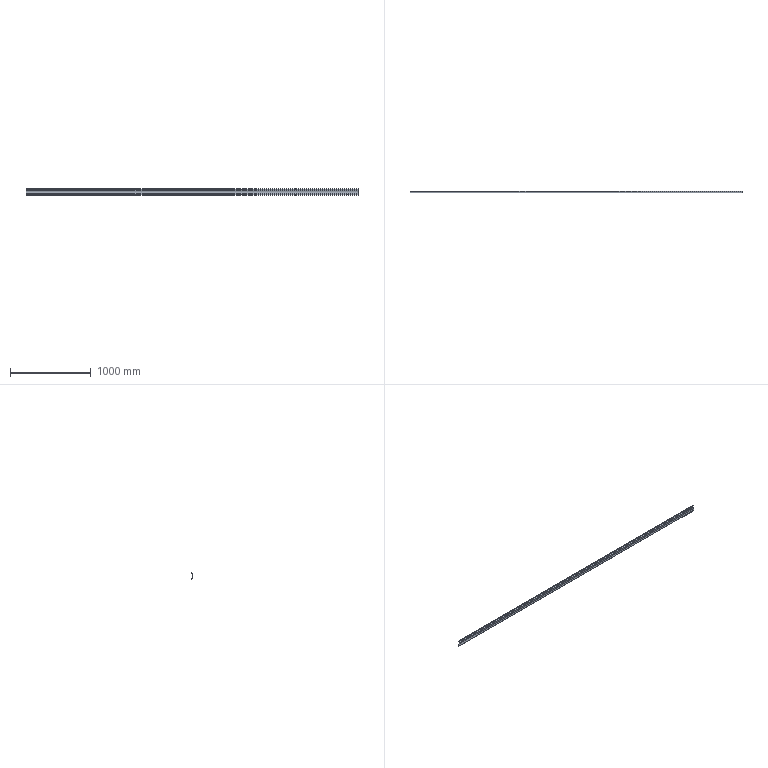Component | SolidWorks | Assembly2-1_WaterproofSlot-1 | 1 solid | 74 faces | volume 690583 mm3 | cylinder 38 | plane 36 | commonest cylinder face diameters 7 x28 3.4 x5 0.4 x5